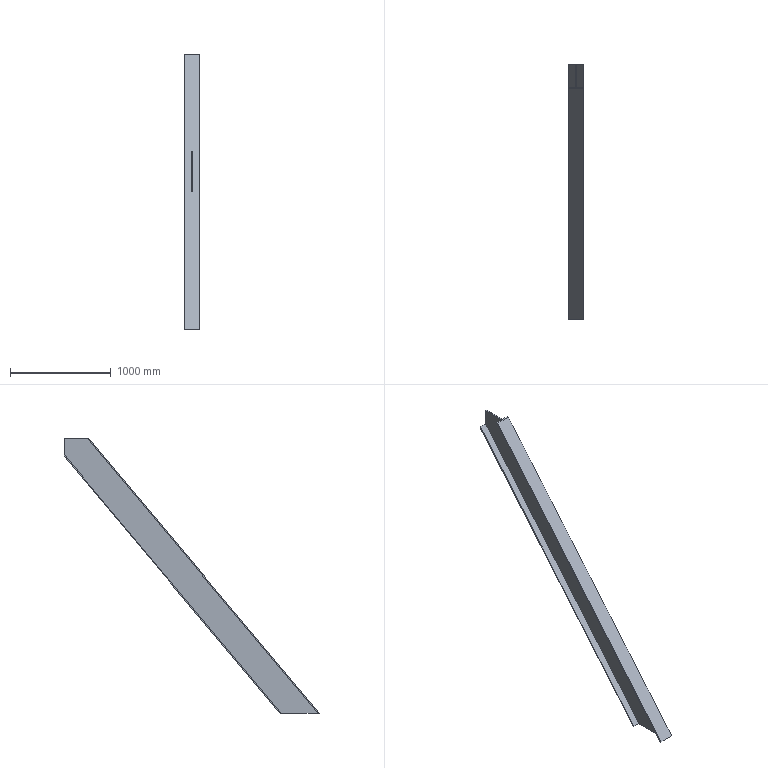Component | NX | ZHIJIA_XIE1 | 1 solid | 15 faces | box 150 x 2527.87 x 2724.41 mm | volume 20181722 mm3 | plane 15
STEP:
#1=CARTESIAN_POINT('',(0.,0.,0.));
#2=DIRECTION('',(0.,0.,1.));
#3=DIRECTION('',(1.,0.,0.));
#4=AXIS2_PLACEMENT_3D('',#1,#2,#3);
#5=CARTESIAN_POINT('',(2505.,2625.,3361.44));
#6=VERTEX_POINT('',#5);
#7=CARTESIAN_POINT('',(2505.,475.697,800.));
#8=VERTEX_POINT('',#7);
#9=CARTESIAN_POINT('',(2505.,2812.666,3585.092));
#10=DIRECTION('',(0.,-0.6428,-0.766));
#11=VECTOR('',#10,1.);
#12=LINE('',#9,#11);
#13=CARTESIAN_POINT('',(2505.,2598.174,3765.072));
#14=DIRECTION('',(-1.,0.,-0.));
#15=DIRECTION('',(-0.,-0.766,0.6428));
#16=AXIS2_PLACEMENT_3D('',#13,#14,#15);
#17=PLANE('',#16);
#18=CARTESIAN_POINT('',(-280.,-0.));
#19=DIRECTION('',(0.,-1.));
#20=VECTOR('',#19,1.);
#21=LINE('',#18,#20);
#22=(GEOMETRIC_REPRESENTATION_CONTEXT(2)PARAMETRIC_REPRESENTATION_CONTEXT()REPRESENTATION_CONTEXT('',''));
#23=DEFINITIONAL_REPRESENTATION('',(#21),#22);
#24=PCURVE('',#17,#23);
#25=CARTESIAN_POINT('',(2505.,2812.666,3585.092));
#26=DIRECTION('',(0.,0.766,-0.6428));
#27=DIRECTION('',(0.,0.6428,0.766));
#28=AXIS2_PLACEMENT_3D('',#25,#26,#27);
#29=PLANE('',#28);
#30=CARTESIAN_POINT('',(0.,0.));
#31=DIRECTION('',(-1.,0.));
#32=VECTOR('',#31,1.);
#33=LINE('',#30,#32);
#34=(GEOMETRIC_REPRESENTATION_CONTEXT(2)PARAMETRIC_REPRESENTATION_CONTEXT()REPRESENTATION_CONTEXT('',''));
#35=DEFINITIONAL_REPRESENTATION('',(#33),#34);
#36=PCURVE('',#29,#35);
#37=SURFACE_CURVE('',#12,(#24,#36),.PCURVE_S1.);
#38=EDGE_CURVE('',#6,#8,#37,.T.);
#39=ORIENTED_EDGE('',*,*,#38,.F.);
#40=CARTESIAN_POINT('',(2505.,2625.,3524.41));
#41=VERTEX_POINT('',#40);
#42=CARTESIAN_POINT('',(2505.,2625.,3765.072));
#43=DIRECTION('',(-0.,-0.,1.));
#44=VECTOR('',#43,1.);
#45=LINE('',#42,#44);
#46=CARTESIAN_POINT('',(-20.55,17.244));
#47=DIRECTION('',(0.6428,0.766));
#48=VECTOR('',#47,1.);
#49=LINE('',#46,#48);
#50=(GEOMETRIC_REPRESENTATION_CONTEXT(2)PARAMETRIC_REPRESENTATION_CONTEXT()REPRESENTATION_CONTEXT('',''));
#51=DEFINITIONAL_REPRESENTATION('',(#49),#50);
#52=PCURVE('',#17,#51);
#53=CARTESIAN_POINT('',(9500.,2625.,3117.693));
#54=DIRECTION('',(0.,-1.,-0.));
#55=DIRECTION('',(0.,0.,-1.));
#56=AXIS2_PLACEMENT_3D('',#53,#54,#55);
#57=PLANE('',#56);
#58=CARTESIAN_POINT('',(-647.379,-6995.));
#59=DIRECTION('',(-1.,-0.));
#60=VECTOR('',#59,1.);
#61=LINE('',#58,#60);
#62=(GEOMETRIC_REPRESENTATION_CONTEXT(2)PARAMETRIC_REPRESENTATION_CONTEXT()REPRESENTATION_CONTEXT('',''));
#63=DEFINITIONAL_REPRESENTATION('',(#61),#62);
#64=PCURVE('',#57,#63);
#65=SURFACE_CURVE('',#45,(#52,#64),.PCURVE_S1.);
#66=EDGE_CURVE('',#6,#41,#65,.T.);
#67=ORIENTED_EDGE('',*,*,#66,.T.);
#68=CARTESIAN_POINT('',(2505.,2396.234,3524.41));
#69=VERTEX_POINT('',#68);
#70=CARTESIAN_POINT('',(2505.,2598.174,3524.41));
#71=DIRECTION('',(-0.,-1.,0.));
#72=VECTOR('',#71,1.);
#73=LINE('',#70,#72);
#74=CARTESIAN_POINT('',(-154.695,-184.358));
#75=DIRECTION('',(0.766,-0.6428));
#76=VECTOR('',#75,1.);
#77=LINE('',#74,#76);
#78=(GEOMETRIC_REPRESENTATION_CONTEXT(2)PARAMETRIC_REPRESENTATION_CONTEXT()REPRESENTATION_CONTEXT('',''));
#79=DEFINITIONAL_REPRESENTATION('',(#77),#78);
#80=PCURVE('',#17,#79);
#81=CARTESIAN_POINT('',(9500.,2625.,3524.41));
#82=DIRECTION('',(0.,-0.,-1.));
#83=DIRECTION('',(0.,1.,-0.));
#84=AXIS2_PLACEMENT_3D('',#81,#82,#83);
#85=PLANE('',#84);
#86=CARTESIAN_POINT('',(-26.826,-6995.));
#87=DIRECTION('',(-1.,-0.));
#88=VECTOR('',#87,1.);
#89=LINE('',#86,#88);
#90=(GEOMETRIC_REPRESENTATION_CONTEXT(2)PARAMETRIC_REPRESENTATION_CONTEXT()REPRESENTATION_CONTEXT('',''));
#91=DEFINITIONAL_REPRESENTATION('',(#89),#90);
#92=PCURVE('',#85,#91);
#93=SURFACE_CURVE('',#73,(#80,#92),.PCURVE_S1.);
#94=EDGE_CURVE('',#41,#69,#93,.T.);
#95=ORIENTED_EDGE('',*,*,#94,.T.);
#96=CARTESIAN_POINT('',(2505.,110.183,800.));
#97=VERTEX_POINT('',#96);
#98=CARTESIAN_POINT('',(2505.,2598.174,3765.072));
#99=DIRECTION('',(0.,-0.6428,-0.766));
#100=VECTOR('',#99,1.);
#101=LINE('',#98,#100);
#102=CARTESIAN_POINT('',(0.,0.));
#103=DIRECTION('',(0.,-1.));
#104=VECTOR('',#103,1.);
#105=LINE('',#102,#104);
#106=(GEOMETRIC_REPRESENTATION_CONTEXT(2)PARAMETRIC_REPRESENTATION_CONTEXT()REPRESENTATION_CONTEXT('',''));
#107=DEFINITIONAL_REPRESENTATION('',(#105),#106);
#108=PCURVE('',#17,#107);
#109=CARTESIAN_POINT('',(2575.,2598.174,3765.072));
#110=DIRECTION('',(0.,-0.766,0.6428));
#111=DIRECTION('',(0.,-0.6428,-0.766));
#112=AXIS2_PLACEMENT_3D('',#109,#110,#111);
#113=PLANE('',#112);
#114=CARTESIAN_POINT('',(0.,-70.));
#115=DIRECTION('',(1.,0.));
#116=VECTOR('',#115,1.);
#117=LINE('',#114,#116);
#118=(GEOMETRIC_REPRESENTATION_CONTEXT(2)PARAMETRIC_REPRESENTATION_CONTEXT()REPRESENTATION_CONTEXT('',''));
#119=DEFINITIONAL_REPRESENTATION('',(#117),#118);
#120=PCURVE('',#113,#119);
#121=SURFACE_CURVE('',#101,(#108,#120),.PCURVE_S1.);
#122=EDGE_CURVE('',#69,#97,#121,.T.);
#123=ORIENTED_EDGE('',*,*,#122,.T.);
#124=CARTESIAN_POINT('',(2505.,2598.174,800.));
#125=DIRECTION('',(-0.,-1.,-0.));
#126=VECTOR('',#125,1.);
#127=LINE('',#124,#126);
#128=CARTESIAN_POINT('',(-1905.912,-2271.377));
#129=DIRECTION('',(0.766,-0.6428));
#130=VECTOR('',#129,1.);
#131=LINE('',#128,#130);
#132=(GEOMETRIC_REPRESENTATION_CONTEXT(2)PARAMETRIC_REPRESENTATION_CONTEXT()REPRESENTATION_CONTEXT('',''));
#133=DEFINITIONAL_REPRESENTATION('',(#131),#132);
#134=PCURVE('',#17,#133);
#135=CARTESIAN_POINT('',(9500.,631.661,800.));
#136=DIRECTION('',(0.,0.,-1.));
#137=DIRECTION('',(0.,1.,0.));
#138=AXIS2_PLACEMENT_3D('',#135,#136,#137);
#139=PLANE('',#138);
#140=CARTESIAN_POINT('',(1966.512,-6995.));
#141=DIRECTION('',(-1.,-0.));
#142=VECTOR('',#141,1.);
#143=LINE('',#140,#142);
#144=(GEOMETRIC_REPRESENTATION_CONTEXT(2)PARAMETRIC_REPRESENTATION_CONTEXT()REPRESENTATION_CONTEXT('',''));
#145=DEFINITIONAL_REPRESENTATION('',(#143),#144);
#146=PCURVE('',#139,#145);
#147=SURFACE_CURVE('',#127,(#134,#146),.PCURVE_S1.);
#148=EDGE_CURVE('',#8,#97,#147,.T.);
#149=ORIENTED_EDGE('',*,*,#148,.F.);
#150=EDGE_LOOP('',(#39,#67,#95,#123,#149));
#151=FACE_BOUND('',#150,.T.);
#152=ADVANCED_FACE('',(#151),#17,.F.);
#153=CARTESIAN_POINT('',(2575.,2625.,3361.44));
#154=VERTEX_POINT('',#153);
#155=CARTESIAN_POINT('',(2575.,475.697,800.));
#156=VERTEX_POINT('',#155);
#157=CARTESIAN_POINT('',(2575.,2812.666,3585.092));
#158=DIRECTION('',(0.,-0.6428,-0.766));
#159=VECTOR('',#158,1.);
#160=LINE('',#157,#159);
#161=CARTESIAN_POINT('',(0.,70.));
#162=DIRECTION('',(-1.,0.));
#163=VECTOR('',#162,1.);
#164=LINE('',#161,#163);
#165=(GEOMETRIC_REPRESENTATION_CONTEXT(2)PARAMETRIC_REPRESENTATION_CONTEXT()REPRESENTATION_CONTEXT('',''));
#166=DEFINITIONAL_REPRESENTATION('',(#164),#165);
#167=PCURVE('',#29,#166);
#168=CARTESIAN_POINT('',(2575.,2812.666,3585.092));
#169=DIRECTION('',(-1.,0.,-0.));
#170=DIRECTION('',(-0.,-0.766,0.6428));
#171=AXIS2_PLACEMENT_3D('',#168,#169,#170);
#172=PLANE('',#171);
#173=CARTESIAN_POINT('',(0.,0.));
#174=DIRECTION('',(0.,-1.));
#175=VECTOR('',#174,1.);
#176=LINE('',#173,#175);
#177=(GEOMETRIC_REPRESENTATION_CONTEXT(2)PARAMETRIC_REPRESENTATION_CONTEXT()REPRESENTATION_CONTEXT('',''));
#178=DEFINITIONAL_REPRESENTATION('',(#176),#177);
#179=PCURVE('',#172,#178);
#180=SURFACE_CURVE('',#160,(#167,#179),.PCURVE_S1.);
#181=EDGE_CURVE('',#154,#156,#180,.T.);
#182=ORIENTED_EDGE('',*,*,#181,.F.);
#183=CARTESIAN_POINT('',(2505.,2625.,3361.44));
#184=DIRECTION('',(-1.,0.,0.));
#185=VECTOR('',#184,1.);
#186=LINE('',#183,#185);
#187=CARTESIAN_POINT('',(-291.957,0.));
#188=DIRECTION('',(0.,-1.));
#189=VECTOR('',#188,1.);
#190=LINE('',#187,#189);
#191=(GEOMETRIC_REPRESENTATION_CONTEXT(2)PARAMETRIC_REPRESENTATION_CONTEXT()REPRESENTATION_CONTEXT('',''));
#192=DEFINITIONAL_REPRESENTATION('',(#190),#191);
#193=PCURVE('',#29,#192);
#194=CARTESIAN_POINT('',(-243.747,-6995.));
#195=DIRECTION('',(0.,-1.));
#196=VECTOR('',#195,1.);
#197=LINE('',#194,#196);
#198=(GEOMETRIC_REPRESENTATION_CONTEXT(2)PARAMETRIC_REPRESENTATION_CONTEXT()REPRESENTATION_CONTEXT('',''));
#199=DEFINITIONAL_REPRESENTATION('',(#197),#198);
#200=PCURVE('',#57,#199);
#201=SURFACE_CURVE('',#186,(#193,#200),.PCURVE_S1.);
#202=EDGE_CURVE('',#154,#6,#201,.T.);
#203=ORIENTED_EDGE('',*,*,#202,.T.);
#204=ORIENTED_EDGE('',*,*,#38,.T.);
#205=CARTESIAN_POINT('',(2505.,475.697,800.));
#206=DIRECTION('',(-1.,0.,0.));
#207=VECTOR('',#206,1.);
#208=LINE('',#205,#207);
#209=CARTESIAN_POINT('',(-3635.679,0.));
#210=DIRECTION('',(0.,-1.));
#211=VECTOR('',#210,1.);
#212=LINE('',#209,#211);
#213=(GEOMETRIC_REPRESENTATION_CONTEXT(2)PARAMETRIC_REPRESENTATION_CONTEXT()REPRESENTATION_CONTEXT('',''));
#214=DEFINITIONAL_REPRESENTATION('',(#212),#213);
#215=PCURVE('',#29,#214);
#216=CARTESIAN_POINT('',(-155.965,-6995.));
#217=DIRECTION('',(0.,-1.));
#218=VECTOR('',#217,1.);
#219=LINE('',#216,#218);
#220=(GEOMETRIC_REPRESENTATION_CONTEXT(2)PARAMETRIC_REPRESENTATION_CONTEXT()REPRESENTATION_CONTEXT('',''));
#221=DEFINITIONAL_REPRESENTATION('',(#219),#220);
#222=PCURVE('',#139,#221);
#223=SURFACE_CURVE('',#208,(#215,#222),.PCURVE_S1.);
#224=EDGE_CURVE('',#156,#8,#223,.T.);
#225=ORIENTED_EDGE('',*,*,#224,.F.);
#226=EDGE_LOOP('',(#182,#203,#204,#225));
#227=FACE_BOUND('',#226,.T.);
#228=ADVANCED_FACE('',(#227),#29,.F.);
#229=CARTESIAN_POINT('',(2575.,2625.,3345.883));
#230=VERTEX_POINT('',#229);
#231=CARTESIAN_POINT('',(2575.,488.751,800.));
#232=VERTEX_POINT('',#231);
#233=CARTESIAN_POINT('',(2575.,2820.327,3578.664));
#234=DIRECTION('',(0.,-0.6428,-0.766));
#235=VECTOR('',#234,1.);
#236=LINE('',#233,#235);
#237=CARTESIAN_POINT('',(-10.,0.));
#238=DIRECTION('',(0.,-1.));
#239=VECTOR('',#238,1.);
#240=LINE('',#237,#239);
#241=(GEOMETRIC_REPRESENTATION_CONTEXT(2)PARAMETRIC_REPRESENTATION_CONTEXT()REPRESENTATION_CONTEXT('',''));
#242=DEFINITIONAL_REPRESENTATION('',(#240),#241);
#243=PCURVE('',#172,#242);
#244=CARTESIAN_POINT('',(2575.,2820.327,3578.664));
#245=DIRECTION('',(0.,-0.766,0.6428));
#246=DIRECTION('',(0.,-0.6428,-0.766));
#247=AXIS2_PLACEMENT_3D('',#244,#245,#246);
#248=PLANE('',#247);
#249=CARTESIAN_POINT('',(0.,0.));
#250=DIRECTION('',(1.,0.));
#251=VECTOR('',#250,1.);
#252=LINE('',#249,#251);
#253=(GEOMETRIC_REPRESENTATION_CONTEXT(2)PARAMETRIC_REPRESENTATION_CONTEXT()REPRESENTATION_CONTEXT('',''));
#254=DEFINITIONAL_REPRESENTATION('',(#252),#253);
#255=PCURVE('',#248,#254);
#256=SURFACE_CURVE('',#236,(#243,#255),.PCURVE_S1.);
#257=EDGE_CURVE('',#230,#232,#256,.T.);
#258=ORIENTED_EDGE('',*,*,#257,.F.);
#259=CARTESIAN_POINT('',(2575.,2625.,3585.092));
#260=DIRECTION('',(-0.,-0.,1.));
#261=VECTOR('',#260,1.);
#262=LINE('',#259,#261);
#263=CARTESIAN_POINT('',(143.761,-120.63));
#264=DIRECTION('',(0.6428,0.766));
#265=VECTOR('',#264,1.);
#266=LINE('',#263,#265);
#267=(GEOMETRIC_REPRESENTATION_CONTEXT(2)PARAMETRIC_REPRESENTATION_CONTEXT()REPRESENTATION_CONTEXT('',''));
#268=DEFINITIONAL_REPRESENTATION('',(#266),#267);
#269=PCURVE('',#172,#268);
#270=CARTESIAN_POINT('',(-467.399,-6925.));
#271=DIRECTION('',(-1.,-0.));
#272=VECTOR('',#271,1.);
#273=LINE('',#270,#272);
#274=(GEOMETRIC_REPRESENTATION_CONTEXT(2)PARAMETRIC_REPRESENTATION_CONTEXT()REPRESENTATION_CONTEXT('',''));
#275=DEFINITIONAL_REPRESENTATION('',(#273),#274);
#276=PCURVE('',#57,#275);
#277=SURFACE_CURVE('',#262,(#269,#276),.PCURVE_S1.);
#278=EDGE_CURVE('',#230,#154,#277,.T.);
#279=ORIENTED_EDGE('',*,*,#278,.T.);
#280=ORIENTED_EDGE('',*,*,#181,.T.);
#281=CARTESIAN_POINT('',(2575.,2812.666,800.));
#282=DIRECTION('',(-0.,-1.,-0.));
#283=VECTOR('',#282,1.);
#284=LINE('',#281,#283);
#285=CARTESIAN_POINT('',(-1790.223,-2133.504));
#286=DIRECTION('',(0.766,-0.6428));
#287=VECTOR('',#286,1.);
#288=LINE('',#285,#287);
#289=(GEOMETRIC_REPRESENTATION_CONTEXT(2)PARAMETRIC_REPRESENTATION_CONTEXT()REPRESENTATION_CONTEXT('',''));
#290=DEFINITIONAL_REPRESENTATION('',(#288),#289);
#291=PCURVE('',#172,#290);
#292=CARTESIAN_POINT('',(2181.005,-6925.));
#293=DIRECTION('',(-1.,-0.));
#294=VECTOR('',#293,1.);
#295=LINE('',#292,#294);
#296=(GEOMETRIC_REPRESENTATION_CONTEXT(2)PARAMETRIC_REPRESENTATION_CONTEXT()REPRESENTATION_CONTEXT('',''));
#297=DEFINITIONAL_REPRESENTATION('',(#295),#296);
#298=PCURVE('',#139,#297);
#299=SURFACE_CURVE('',#284,(#291,#298),.PCURVE_S1.);
#300=EDGE_CURVE('',#232,#156,#299,.T.);
#301=ORIENTED_EDGE('',*,*,#300,.F.);
#302=EDGE_LOOP('',(#258,#279,#280,#301));
#303=FACE_BOUND('',#302,.T.);
#304=ADVANCED_FACE('',(#303),#172,.F.);
#305=CARTESIAN_POINT('',(2425.,2625.,3345.883));
#306=VERTEX_POINT('',#305);
#307=CARTESIAN_POINT('',(2425.,488.751,800.));
#308=VERTEX_POINT('',#307);
#309=CARTESIAN_POINT('',(2425.,2820.327,3578.664));
#310=DIRECTION('',(0.,-0.6428,-0.766));
#311=VECTOR('',#310,1.);
#312=LINE('',#309,#311);
#313=CARTESIAN_POINT('',(0.,-150.));
#314=DIRECTION('',(1.,0.));
#315=VECTOR('',#314,1.);
#316=LINE('',#313,#315);
#317=(GEOMETRIC_REPRESENTATION_CONTEXT(2)PARAMETRIC_REPRESENTATION_CONTEXT()REPRESENTATION_CONTEXT('',''));
#318=DEFINITIONAL_REPRESENTATION('',(#316),#317);
#319=PCURVE('',#248,#318);
#320=CARTESIAN_POINT('',(2425.,2820.327,3578.664));
#321=DIRECTION('',(1.,-0.,0.));
#322=DIRECTION('',(0.,0.766,-0.6428));
#323=AXIS2_PLACEMENT_3D('',#320,#321,#322);
#324=PLANE('',#323);
#325=CARTESIAN_POINT('',(0.,0.));
#326=DIRECTION('',(0.,-1.));
#327=VECTOR('',#326,1.);
#328=LINE('',#325,#327);
#329=(GEOMETRIC_REPRESENTATION_CONTEXT(2)PARAMETRIC_REPRESENTATION_CONTEXT()REPRESENTATION_CONTEXT('',''));
#330=DEFINITIONAL_REPRESENTATION('',(#328),#329);
#331=PCURVE('',#324,#330);
#332=SURFACE_CURVE('',#312,(#319,#331),.PCURVE_S1.);
#333=EDGE_CURVE('',#306,#308,#332,.T.);
#334=ORIENTED_EDGE('',*,*,#333,.F.);
#335=CARTESIAN_POINT('',(2575.,2625.,3345.883));
#336=DIRECTION('',(1.,0.,0.));
#337=VECTOR('',#336,1.);
#338=LINE('',#335,#337);
#339=CARTESIAN_POINT('',(303.874,0.));
#340=DIRECTION('',(0.,1.));
#341=VECTOR('',#340,1.);
#342=LINE('',#339,#341);
#343=(GEOMETRIC_REPRESENTATION_CONTEXT(2)PARAMETRIC_REPRESENTATION_CONTEXT()REPRESENTATION_CONTEXT('',''));
#344=DEFINITIONAL_REPRESENTATION('',(#342),#343);
#345=PCURVE('',#248,#344);
#346=CARTESIAN_POINT('',(-228.19,-6925.));
#347=DIRECTION('',(0.,1.));
#348=VECTOR('',#347,1.);
#349=LINE('',#346,#348);
#350=(GEOMETRIC_REPRESENTATION_CONTEXT(2)PARAMETRIC_REPRESENTATION_CONTEXT()REPRESENTATION_CONTEXT('',''));
#351=DEFINITIONAL_REPRESENTATION('',(#349),#350);
#352=PCURVE('',#57,#351);
#353=SURFACE_CURVE('',#338,(#345,#352),.PCURVE_S1.);
#354=EDGE_CURVE('',#306,#230,#353,.T.);
#355=ORIENTED_EDGE('',*,*,#354,.T.);
#356=ORIENTED_EDGE('',*,*,#257,.T.);
#357=CARTESIAN_POINT('',(2575.,488.751,800.));
#358=DIRECTION('',(1.,0.,0.));
#359=VECTOR('',#358,1.);
#360=LINE('',#357,#359);
#361=CARTESIAN_POINT('',(3627.288,0.));
#362=DIRECTION('',(0.,1.));
#363=VECTOR('',#362,1.);
#364=LINE('',#361,#363);
#365=(GEOMETRIC_REPRESENTATION_CONTEXT(2)PARAMETRIC_REPRESENTATION_CONTEXT()REPRESENTATION_CONTEXT('',''));
#366=DEFINITIONAL_REPRESENTATION('',(#364),#365);
#367=PCURVE('',#248,#366);
#368=CARTESIAN_POINT('',(-142.911,-6925.));
#369=DIRECTION('',(0.,1.));
#370=VECTOR('',#369,1.);
#371=LINE('',#368,#370);
#372=(GEOMETRIC_REPRESENTATION_CONTEXT(2)PARAMETRIC_REPRESENTATION_CONTEXT()REPRESENTATION_CONTEXT('',''));
#373=DEFINITIONAL_REPRESENTATION('',(#371),#372);
#374=PCURVE('',#139,#373);
#375=SURFACE_CURVE('',#360,(#367,#374),.PCURVE_S1.);
#376=EDGE_CURVE('',#308,#232,#375,.T.);
#377=ORIENTED_EDGE('',*,*,#376,.F.);
#378=EDGE_LOOP('',(#334,#355,#356,#377));
#379=FACE_BOUND('',#378,.T.);
#380=ADVANCED_FACE('',(#379),#248,.F.);
#381=CARTESIAN_POINT('',(2425.,2625.,3361.44));
#382=VERTEX_POINT('',#381);
#383=CARTESIAN_POINT('',(2425.,475.697,800.));
#384=VERTEX_POINT('',#383);
#385=CARTESIAN_POINT('',(2425.,2812.666,3585.092));
#386=DIRECTION('',(0.,-0.6428,-0.766));
#387=VECTOR('',#386,1.);
#388=LINE('',#385,#387);
#389=CARTESIAN_POINT('',(-10.,-0.));
#390=DIRECTION('',(0.,-1.));
#391=VECTOR('',#390,1.);
#392=LINE('',#389,#391);
#393=(GEOMETRIC_REPRESENTATION_CONTEXT(2)PARAMETRIC_REPRESENTATION_CONTEXT()REPRESENTATION_CONTEXT('',''));
#394=DEFINITIONAL_REPRESENTATION('',(#392),#393);
#395=PCURVE('',#324,#394);
#396=CARTESIAN_POINT('',(2425.,2812.666,3585.092));
#397=DIRECTION('',(0.,0.766,-0.6428));
#398=DIRECTION('',(0.,0.6428,0.766));
#399=AXIS2_PLACEMENT_3D('',#396,#397,#398);
#400=PLANE('',#399);
#401=CARTESIAN_POINT('',(0.,0.));
#402=DIRECTION('',(-1.,0.));
#403=VECTOR('',#402,1.);
#404=LINE('',#401,#403);
#405=(GEOMETRIC_REPRESENTATION_CONTEXT(2)PARAMETRIC_REPRESENTATION_CONTEXT()REPRESENTATION_CONTEXT('',''));
#406=DEFINITIONAL_REPRESENTATION('',(#404),#405);
#407=PCURVE('',#400,#406);
#408=SURFACE_CURVE('',#388,(#395,#407),.PCURVE_S1.);
#409=EDGE_CURVE('',#382,#384,#408,.T.);
#410=ORIENTED_EDGE('',*,*,#409,.F.);
#411=CARTESIAN_POINT('',(2425.,2625.,3578.664));
#412=DIRECTION('',(0.,0.,-1.));
#413=VECTOR('',#412,1.);
#414=LINE('',#411,#413);
#415=CARTESIAN_POINT('',(-149.629,-125.554));
#416=DIRECTION('',(0.6428,-0.766));
#417=VECTOR('',#416,1.);
#418=LINE('',#415,#417);
#419=(GEOMETRIC_REPRESENTATION_CONTEXT(2)PARAMETRIC_REPRESENTATION_CONTEXT()REPRESENTATION_CONTEXT('',''));
#420=DEFINITIONAL_REPRESENTATION('',(#418),#419);
#421=PCURVE('',#324,#420);
#422=CARTESIAN_POINT('',(-460.971,-7075.));
#423=DIRECTION('',(1.,0.));
#424=VECTOR('',#423,1.);
#425=LINE('',#422,#424);
#426=(GEOMETRIC_REPRESENTATION_CONTEXT(2)PARAMETRIC_REPRESENTATION_CONTEXT()REPRESENTATION_CONTEXT('',''));
#427=DEFINITIONAL_REPRESENTATION('',(#425),#426);
#428=PCURVE('',#57,#427);
#429=SURFACE_CURVE('',#414,(#421,#428),.PCURVE_S1.);
#430=EDGE_CURVE('',#382,#306,#429,.T.);
#431=ORIENTED_EDGE('',*,*,#430,.T.);
#432=ORIENTED_EDGE('',*,*,#333,.T.);
#433=CARTESIAN_POINT('',(2425.,2820.327,800.));
#434=DIRECTION('',(0.,1.,0.));
#435=VECTOR('',#434,1.);
#436=LINE('',#433,#435);
#437=CARTESIAN_POINT('',(1786.091,-2128.58));
#438=DIRECTION('',(0.766,0.6428));
#439=VECTOR('',#438,1.);
#440=LINE('',#437,#439);
#441=(GEOMETRIC_REPRESENTATION_CONTEXT(2)PARAMETRIC_REPRESENTATION_CONTEXT()REPRESENTATION_CONTEXT('',''));
#442=DEFINITIONAL_REPRESENTATION('',(#440),#441);
#443=PCURVE('',#324,#442);
#444=CARTESIAN_POINT('',(2188.665,-7075.));
#445=DIRECTION('',(1.,0.));
#446=VECTOR('',#445,1.);
#447=LINE('',#444,#446);
#448=(GEOMETRIC_REPRESENTATION_CONTEXT(2)PARAMETRIC_REPRESENTATION_CONTEXT()REPRESENTATION_CONTEXT('',''));
#449=DEFINITIONAL_REPRESENTATION('',(#447),#448);
#450=PCURVE('',#139,#449);
#451=SURFACE_CURVE('',#436,(#443,#450),.PCURVE_S1.);
#452=EDGE_CURVE('',#384,#308,#451,.T.);
#453=ORIENTED_EDGE('',*,*,#452,.F.);
#454=EDGE_LOOP('',(#410,#431,#432,#453));
#455=FACE_BOUND('',#454,.T.);
#456=ADVANCED_FACE('',(#455),#324,.F.);
#457=CARTESIAN_POINT('',(2495.,2625.,3361.44));
#458=VERTEX_POINT('',#457);
#459=CARTESIAN_POINT('',(2495.,475.697,800.));
#460=VERTEX_POINT('',#459);
#461=CARTESIAN_POINT('',(2495.,2812.666,3585.092));
#462=DIRECTION('',(0.,-0.6428,-0.766));
#463=VECTOR('',#462,1.);
#464=LINE('',#461,#463);
#465=CARTESIAN_POINT('',(0.,70.));
#466=DIRECTION('',(-1.,0.));
#467=VECTOR('',#466,1.);
#468=LINE('',#465,#467);
#469=(GEOMETRIC_REPRESENTATION_CONTEXT(2)PARAMETRIC_REPRESENTATION_CONTEXT()REPRESENTATION_CONTEXT('',''));
#470=DEFINITIONAL_REPRESENTATION('',(#468),#469);
#471=PCURVE('',#400,#470);
#472=CARTESIAN_POINT('',(2495.,2812.666,3585.092));
#473=DIRECTION('',(1.,-0.,0.));
#474=DIRECTION('',(0.,0.766,-0.6428));
#475=AXIS2_PLACEMENT_3D('',#472,#473,#474);
#476=PLANE('',#475);
#477=CARTESIAN_POINT('',(0.,0.));
#478=DIRECTION('',(0.,-1.));
#479=VECTOR('',#478,1.);
#480=LINE('',#477,#479);
#481=(GEOMETRIC_REPRESENTATION_CONTEXT(2)PARAMETRIC_REPRESENTATION_CONTEXT()REPRESENTATION_CONTEXT('',''));
#482=DEFINITIONAL_REPRESENTATION('',(#480),#481);
#483=PCURVE('',#476,#482);
#484=SURFACE_CURVE('',#464,(#471,#483),.PCURVE_S1.);
#485=EDGE_CURVE('',#458,#460,#484,.T.);
#486=ORIENTED_EDGE('',*,*,#485,.F.);
#487=CARTESIAN_POINT('',(2425.,2625.,3361.44));
#488=DIRECTION('',(-1.,0.,0.));
#489=VECTOR('',#488,1.);
#490=LINE('',#487,#489);
#491=CARTESIAN_POINT('',(-291.957,0.));
#492=DIRECTION('',(0.,-1.));
#493=VECTOR('',#492,1.);
#494=LINE('',#491,#493);
#495=(GEOMETRIC_REPRESENTATION_CONTEXT(2)PARAMETRIC_REPRESENTATION_CONTEXT()REPRESENTATION_CONTEXT('',''));
#496=DEFINITIONAL_REPRESENTATION('',(#494),#495);
#497=PCURVE('',#400,#496);
#498=CARTESIAN_POINT('',(-243.747,-7075.));
#499=DIRECTION('',(0.,-1.));
#500=VECTOR('',#499,1.);
#501=LINE('',#498,#500);
#502=(GEOMETRIC_REPRESENTATION_CONTEXT(2)PARAMETRIC_REPRESENTATION_CONTEXT()REPRESENTATION_CONTEXT('',''));
#503=DEFINITIONAL_REPRESENTATION('',(#501),#502);
#504=PCURVE('',#57,#503);
#505=SURFACE_CURVE('',#490,(#497,#504),.PCURVE_S1.);
#506=EDGE_CURVE('',#458,#382,#505,.T.);
#507=ORIENTED_EDGE('',*,*,#506,.T.);
#508=ORIENTED_EDGE('',*,*,#409,.T.);
#509=CARTESIAN_POINT('',(2425.,475.697,800.));
#510=DIRECTION('',(-1.,0.,0.));
#511=VECTOR('',#510,1.);
#512=LINE('',#509,#511);
#513=CARTESIAN_POINT('',(-3635.679,0.));
#514=DIRECTION('',(0.,-1.));
#515=VECTOR('',#514,1.);
#516=LINE('',#513,#515);
#517=(GEOMETRIC_REPRESENTATION_CONTEXT(2)PARAMETRIC_REPRESENTATION_CONTEXT()REPRESENTATION_CONTEXT('',''));
#518=DEFINITIONAL_REPRESENTATION('',(#516),#517);
#519=PCURVE('',#400,#518);
#520=CARTESIAN_POINT('',(-155.965,-7075.));
#521=DIRECTION('',(0.,-1.));
#522=VECTOR('',#521,1.);
#523=LINE('',#520,#522);
#524=(GEOMETRIC_REPRESENTATION_CONTEXT(2)PARAMETRIC_REPRESENTATION_CONTEXT()REPRESENTATION_CONTEXT('',''));
#525=DEFINITIONAL_REPRESENTATION('',(#523),#524);
#526=PCURVE('',#139,#525);
#527=SURFACE_CURVE('',#512,(#519,#526),.PCURVE_S1.);
#528=EDGE_CURVE('',#460,#384,#527,.T.);
#529=ORIENTED_EDGE('',*,*,#528,.F.);
#530=EDGE_LOOP('',(#486,#507,#508,#529));
#531=FACE_BOUND('',#530,.T.);
#532=ADVANCED_FACE('',(#531),#400,.F.);
#533=CARTESIAN_POINT('',(2495.,2396.234,3524.41));
#534=VERTEX_POINT('',#533);
#535=CARTESIAN_POINT('',(2495.,2625.,3524.41));
#536=VERTEX_POINT('',#535);
#537=CARTESIAN_POINT('',(2495.,2812.666,3524.41));
#538=DIRECTION('',(0.,1.,-0.));
#539=VECTOR('',#538,1.);
#540=LINE('',#537,#539);
#541=CARTESIAN_POINT('',(39.005,-46.485));
#542=DIRECTION('',(0.766,0.6428));
#543=VECTOR('',#542,1.);
#544=LINE('',#541,#543);
#545=(GEOMETRIC_REPRESENTATION_CONTEXT(2)PARAMETRIC_REPRESENTATION_CONTEXT()REPRESENTATION_CONTEXT('',''));
#546=DEFINITIONAL_REPRESENTATION('',(#544),#545);
#547=PCURVE('',#476,#546);
#548=CARTESIAN_POINT('',(187.666,-7005.));
#549=DIRECTION('',(1.,0.));
#550=VECTOR('',#549,1.);
#551=LINE('',#548,#550);
#552=(GEOMETRIC_REPRESENTATION_CONTEXT(2)PARAMETRIC_REPRESENTATION_CONTEXT()REPRESENTATION_CONTEXT('',''));
#553=DEFINITIONAL_REPRESENTATION('',(#551),#552);
#554=PCURVE('',#85,#553);
#555=SURFACE_CURVE('',#540,(#547,#554),.PCURVE_S1.);
#556=EDGE_CURVE('',#534,#536,#555,.T.);
#557=ORIENTED_EDGE('',*,*,#556,.T.);
#558=CARTESIAN_POINT('',(2495.,2625.,3585.092));
#559=DIRECTION('',(0.,0.,-1.));
#560=VECTOR('',#559,1.);
#561=LINE('',#558,#560);
#562=CARTESIAN_POINT('',(-143.761,-120.63));
#563=DIRECTION('',(0.6428,-0.766));
#564=VECTOR('',#563,1.);
#565=LINE('',#562,#564);
#566=(GEOMETRIC_REPRESENTATION_CONTEXT(2)PARAMETRIC_REPRESENTATION_CONTEXT()REPRESENTATION_CONTEXT('',''));
#567=DEFINITIONAL_REPRESENTATION('',(#565),#566);
#568=PCURVE('',#476,#567);
#569=CARTESIAN_POINT('',(-467.399,-7005.));
#570=DIRECTION('',(1.,0.));
#571=VECTOR('',#570,1.);
#572=LINE('',#569,#571);
#573=(GEOMETRIC_REPRESENTATION_CONTEXT(2)PARAMETRIC_REPRESENTATION_CONTEXT()REPRESENTATION_CONTEXT('',''));
#574=DEFINITIONAL_REPRESENTATION('',(#572),#573);
#575=PCURVE('',#57,#574);
#576=SURFACE_CURVE('',#561,(#568,#575),.PCURVE_S1.);
#577=EDGE_CURVE('',#536,#458,#576,.T.);
#578=ORIENTED_EDGE('',*,*,#577,.T.);
#579=ORIENTED_EDGE('',*,*,#485,.T.);
#580=CARTESIAN_POINT('',(2495.,110.183,800.));
#581=VERTEX_POINT('',#580);
#582=CARTESIAN_POINT('',(2495.,2812.666,800.));
#583=DIRECTION('',(0.,1.,0.));
#584=VECTOR('',#583,1.);
#585=LINE('',#582,#584);
#586=CARTESIAN_POINT('',(1790.223,-2133.504));
#587=DIRECTION('',(0.766,0.6428));
#588=VECTOR('',#587,1.);
#589=LINE('',#586,#588);
#590=(GEOMETRIC_REPRESENTATION_CONTEXT(2)PARAMETRIC_REPRESENTATION_CONTEXT()REPRESENTATION_CONTEXT('',''));
#591=DEFINITIONAL_REPRESENTATION('',(#589),#590);
#592=PCURVE('',#476,#591);
#593=CARTESIAN_POINT('',(2181.005,-7005.));
#594=DIRECTION('',(1.,0.));
#595=VECTOR('',#594,1.);
#596=LINE('',#593,#595);
#597=(GEOMETRIC_REPRESENTATION_CONTEXT(2)PARAMETRIC_REPRESENTATION_CONTEXT()REPRESENTATION_CONTEXT('',''));
#598=DEFINITIONAL_REPRESENTATION('',(#596),#597);
#599=PCURVE('',#139,#598);
#600=SURFACE_CURVE('',#585,(#592,#599),.PCURVE_S1.);
#601=EDGE_CURVE('',#581,#460,#600,.T.);
#602=ORIENTED_EDGE('',*,*,#601,.F.);
#603=CARTESIAN_POINT('',(2495.,2598.174,3765.072));
#604=DIRECTION('',(0.,-0.6428,-0.766));
#605=VECTOR('',#604,1.);
#606=LINE('',#603,#605);
#607=CARTESIAN_POINT('',(-280.,0.));
#608=DIRECTION('',(0.,-1.));
#609=VECTOR('',#608,1.);
#610=LINE('',#607,#609);
#611=(GEOMETRIC_REPRESENTATION_CONTEXT(2)PARAMETRIC_REPRESENTATION_CONTEXT()REPRESENTATION_CONTEXT('',''));
#612=DEFINITIONAL_REPRESENTATION('',(#610),#611);
#613=PCURVE('',#476,#612);
#614=CARTESIAN_POINT('',(2495.,2598.174,3765.072));
#615=DIRECTION('',(0.,-0.766,0.6428));
#616=DIRECTION('',(0.,-0.6428,-0.766));
#617=AXIS2_PLACEMENT_3D('',#614,#615,#616);
#618=PLANE('',#617);
#619=CARTESIAN_POINT('',(0.,0.));
#620=DIRECTION('',(1.,0.));
#621=VECTOR('',#620,1.);
#622=LINE('',#619,#621);
#623=(GEOMETRIC_REPRESENTATION_CONTEXT(2)PARAMETRIC_REPRESENTATION_CONTEXT()REPRESENTATION_CONTEXT('',''));
#624=DEFINITIONAL_REPRESENTATION('',(#622),#623);
#625=PCURVE('',#618,#624);
#626=SURFACE_CURVE('',#606,(#613,#625),.PCURVE_S1.);
#627=EDGE_CURVE('',#534,#581,#626,.T.);
#628=ORIENTED_EDGE('',*,*,#627,.F.);
#629=EDGE_LOOP('',(#557,#578,#579,#602,#628));
#630=FACE_BOUND('',#629,.T.);
#631=ADVANCED_FACE('',(#630),#476,.F.);
#632=CARTESIAN_POINT('',(2425.,2396.234,3524.41));
#633=VERTEX_POINT('',#632);
#634=CARTESIAN_POINT('',(2425.,110.183,800.));
#635=VERTEX_POINT('',#634);
#636=CARTESIAN_POINT('',(2425.,2598.174,3765.072));
#637=DIRECTION('',(0.,-0.6428,-0.766));
#638=VECTOR('',#637,1.);
#639=LINE('',#636,#638);
#640=CARTESIAN_POINT('',(0.,-70.));
#641=DIRECTION('',(1.,0.));
#642=VECTOR('',#641,1.);
#643=LINE('',#640,#642);
#644=(GEOMETRIC_REPRESENTATION_CONTEXT(2)PARAMETRIC_REPRESENTATION_CONTEXT()REPRESENTATION_CONTEXT('',''));
#645=DEFINITIONAL_REPRESENTATION('',(#643),#644);
#646=PCURVE('',#618,#645);
#647=CARTESIAN_POINT('',(2425.,2598.174,3765.072));
#648=DIRECTION('',(1.,-0.,0.));
#649=DIRECTION('',(0.,0.766,-0.6428));
#650=AXIS2_PLACEMENT_3D('',#647,#648,#649);
#651=PLANE('',#650);
#652=CARTESIAN_POINT('',(0.,0.));
#653=DIRECTION('',(0.,-1.));
#654=VECTOR('',#653,1.);
#655=LINE('',#652,#654);
#656=(GEOMETRIC_REPRESENTATION_CONTEXT(2)PARAMETRIC_REPRESENTATION_CONTEXT()REPRESENTATION_CONTEXT('',''));
#657=DEFINITIONAL_REPRESENTATION('',(#655),#656);
#658=PCURVE('',#651,#657);
#659=SURFACE_CURVE('',#639,(#646,#658),.PCURVE_S1.);
#660=EDGE_CURVE('',#633,#635,#659,.T.);
#661=ORIENTED_EDGE('',*,*,#660,.F.);
#662=CARTESIAN_POINT('',(2495.,2396.234,3524.41));
#663=DIRECTION('',(1.,0.,0.));
#664=VECTOR('',#663,1.);
#665=LINE('',#662,#664);
#666=CARTESIAN_POINT('',(314.162,0.));
#667=DIRECTION('',(0.,1.));
#668=VECTOR('',#667,1.);
#669=LINE('',#666,#668);
#670=(GEOMETRIC_REPRESENTATION_CONTEXT(2)PARAMETRIC_REPRESENTATION_CONTEXT()REPRESENTATION_CONTEXT('',''));
#671=DEFINITIONAL_REPRESENTATION('',(#669),#670);
#672=PCURVE('',#618,#671);
#673=CARTESIAN_POINT('',(-228.766,-7005.));
#674=DIRECTION('',(0.,1.));
#675=VECTOR('',#674,1.);
#676=LINE('',#673,#675);
#677=(GEOMETRIC_REPRESENTATION_CONTEXT(2)PARAMETRIC_REPRESENTATION_CONTEXT()REPRESENTATION_CONTEXT('',''));
#678=DEFINITIONAL_REPRESENTATION('',(#676),#677);
#679=PCURVE('',#85,#678);
#680=SURFACE_CURVE('',#665,(#672,#679),.PCURVE_S1.);
#681=EDGE_CURVE('',#633,#534,#680,.T.);
#682=ORIENTED_EDGE('',*,*,#681,.T.);
#683=ORIENTED_EDGE('',*,*,#627,.T.);
#684=CARTESIAN_POINT('',(2495.,110.183,800.));
#685=DIRECTION('',(1.,0.,0.));
#686=VECTOR('',#685,1.);
#687=LINE('',#684,#686);
#688=CARTESIAN_POINT('',(3870.627,0.));
#689=DIRECTION('',(0.,1.));
#690=VECTOR('',#689,1.);
#691=LINE('',#688,#690);
#692=(GEOMETRIC_REPRESENTATION_CONTEXT(2)PARAMETRIC_REPRESENTATION_CONTEXT()REPRESENTATION_CONTEXT('',''));
#693=DEFINITIONAL_REPRESENTATION('',(#691),#692);
#694=PCURVE('',#618,#693);
#695=CARTESIAN_POINT('',(-521.479,-7005.));
#696=DIRECTION('',(0.,1.));
#697=VECTOR('',#696,1.);
#698=LINE('',#695,#697);
#699=(GEOMETRIC_REPRESENTATION_CONTEXT(2)PARAMETRIC_REPRESENTATION_CONTEXT()REPRESENTATION_CONTEXT('',''));
#700=DEFINITIONAL_REPRESENTATION('',(#698),#699);
#701=PCURVE('',#139,#700);
#702=SURFACE_CURVE('',#687,(#694,#701),.PCURVE_S1.);
#703=EDGE_CURVE('',#635,#581,#702,.T.);
#704=ORIENTED_EDGE('',*,*,#703,.F.);
#705=EDGE_LOOP('',(#661,#682,#683,#704));
#706=FACE_BOUND('',#705,.T.);
#707=ADVANCED_FACE('',(#706),#618,.F.);
#708=CARTESIAN_POINT('',(2425.,2383.18,3524.41));
#709=VERTEX_POINT('',#708);
#710=CARTESIAN_POINT('',(2425.,97.129,800.));
#711=VERTEX_POINT('',#710);
#712=CARTESIAN_POINT('',(2425.,2590.513,3771.5));
#713=DIRECTION('',(0.,-0.6428,-0.766));
#714=VECTOR('',#713,1.);
#715=LINE('',#712,#714);
#716=CARTESIAN_POINT('',(-10.,0.));
#717=DIRECTION('',(0.,-1.));
#718=VECTOR('',#717,1.);
#719=LINE('',#716,#718);
#720=(GEOMETRIC_REPRESENTATION_CONTEXT(2)PARAMETRIC_REPRESENTATION_CONTEXT()REPRESENTATION_CONTEXT('',''));
#721=DEFINITIONAL_REPRESENTATION('',(#719),#720);
#722=PCURVE('',#651,#721);
#723=CARTESIAN_POINT('',(2425.,2590.513,3771.5));
#724=DIRECTION('',(0.,0.766,-0.6428));
#725=DIRECTION('',(0.,0.6428,0.766));
#726=AXIS2_PLACEMENT_3D('',#723,#724,#725);
#727=PLANE('',#726);
#728=CARTESIAN_POINT('',(0.,0.));
#729=DIRECTION('',(-1.,0.));
#730=VECTOR('',#729,1.);
#731=LINE('',#728,#730);
#732=(GEOMETRIC_REPRESENTATION_CONTEXT(2)PARAMETRIC_REPRESENTATION_CONTEXT()REPRESENTATION_CONTEXT('',''));
#733=DEFINITIONAL_REPRESENTATION('',(#731),#732);
#734=PCURVE('',#727,#733);
#735=SURFACE_CURVE('',#715,(#722,#734),.PCURVE_S1.);
#736=EDGE_CURVE('',#709,#711,#735,.T.);
#737=ORIENTED_EDGE('',*,*,#736,.F.);
#738=CARTESIAN_POINT('',(2425.,2598.174,3524.41));
#739=DIRECTION('',(0.,1.,-0.));
#740=VECTOR('',#739,1.);
#741=LINE('',#738,#740);
#742=CARTESIAN_POINT('',(154.695,-184.358));
#743=DIRECTION('',(0.766,0.6428));
#744=VECTOR('',#743,1.);
#745=LINE('',#742,#744);
#746=(GEOMETRIC_REPRESENTATION_CONTEXT(2)PARAMETRIC_REPRESENTATION_CONTEXT()REPRESENTATION_CONTEXT('',''));
#747=DEFINITIONAL_REPRESENTATION('',(#745),#746);
#748=PCURVE('',#651,#747);
#749=CARTESIAN_POINT('',(-26.826,-7075.));
#750=DIRECTION('',(1.,0.));
#751=VECTOR('',#750,1.);
#752=LINE('',#749,#751);
#753=(GEOMETRIC_REPRESENTATION_CONTEXT(2)PARAMETRIC_REPRESENTATION_CONTEXT()REPRESENTATION_CONTEXT('',''));
#754=DEFINITIONAL_REPRESENTATION('',(#752),#753);
#755=PCURVE('',#85,#754);
#756=SURFACE_CURVE('',#741,(#748,#755),.PCURVE_S1.);
#757=EDGE_CURVE('',#709,#633,#756,.T.);
#758=ORIENTED_EDGE('',*,*,#757,.T.);
#759=ORIENTED_EDGE('',*,*,#660,.T.);
#760=CARTESIAN_POINT('',(2425.,2598.174,800.));
#761=DIRECTION('',(0.,1.,0.));
#762=VECTOR('',#761,1.);
#763=LINE('',#760,#762);
#764=CARTESIAN_POINT('',(1905.912,-2271.377));
#765=DIRECTION('',(0.766,0.6428));
#766=VECTOR('',#765,1.);
#767=LINE('',#764,#766);
#768=(GEOMETRIC_REPRESENTATION_CONTEXT(2)PARAMETRIC_REPRESENTATION_CONTEXT()REPRESENTATION_CONTEXT('',''));
#769=DEFINITIONAL_REPRESENTATION('',(#767),#768);
#770=PCURVE('',#651,#769);
#771=CARTESIAN_POINT('',(1966.512,-7075.));
#772=DIRECTION('',(1.,0.));
#773=VECTOR('',#772,1.);
#774=LINE('',#771,#773);
#775=(GEOMETRIC_REPRESENTATION_CONTEXT(2)PARAMETRIC_REPRESENTATION_CONTEXT()REPRESENTATION_CONTEXT('',''));
#776=DEFINITIONAL_REPRESENTATION('',(#774),#775);
#777=PCURVE('',#139,#776);
#778=SURFACE_CURVE('',#763,(#770,#777),.PCURVE_S1.);
#779=EDGE_CURVE('',#711,#635,#778,.T.);
#780=ORIENTED_EDGE('',*,*,#779,.F.);
#781=EDGE_LOOP('',(#737,#758,#759,#780));
#782=FACE_BOUND('',#781,.T.);
#783=ADVANCED_FACE('',(#782),#651,.F.);
#784=CARTESIAN_POINT('',(2575.,2383.18,3524.41));
#785=VERTEX_POINT('',#784);
#786=CARTESIAN_POINT('',(2575.,97.129,800.));
#787=VERTEX_POINT('',#786);
#788=CARTESIAN_POINT('',(2575.,2590.513,3771.5));
#789=DIRECTION('',(0.,-0.6428,-0.766));
#790=VECTOR('',#789,1.);
#791=LINE('',#788,#790);
#792=CARTESIAN_POINT('',(0.,150.));
#793=DIRECTION('',(-1.,0.));
#794=VECTOR('',#793,1.);
#795=LINE('',#792,#794);
#796=(GEOMETRIC_REPRESENTATION_CONTEXT(2)PARAMETRIC_REPRESENTATION_CONTEXT()REPRESENTATION_CONTEXT('',''));
#797=DEFINITIONAL_REPRESENTATION('',(#795),#796);
#798=PCURVE('',#727,#797);
#799=CARTESIAN_POINT('',(2575.,2590.513,3771.5));
#800=DIRECTION('',(-1.,0.,-0.));
#801=DIRECTION('',(-0.,-0.766,0.6428));
#802=AXIS2_PLACEMENT_3D('',#799,#800,#801);
#803=PLANE('',#802);
#804=CARTESIAN_POINT('',(0.,0.));
#805=DIRECTION('',(0.,-1.));
#806=VECTOR('',#805,1.);
#807=LINE('',#804,#806);
#808=(GEOMETRIC_REPRESENTATION_CONTEXT(2)PARAMETRIC_REPRESENTATION_CONTEXT()REPRESENTATION_CONTEXT('',''));
#809=DEFINITIONAL_REPRESENTATION('',(#807),#808);
#810=PCURVE('',#803,#809);
#811=SURFACE_CURVE('',#791,(#798,#810),.PCURVE_S1.);
#812=EDGE_CURVE('',#785,#787,#811,.T.);
#813=ORIENTED_EDGE('',*,*,#812,.F.);
#814=CARTESIAN_POINT('',(2425.,2383.18,3524.41));
#815=DIRECTION('',(-1.,0.,0.));
#816=VECTOR('',#815,1.);
#817=LINE('',#814,#816);
#818=CARTESIAN_POINT('',(-322.553,0.));
#819=DIRECTION('',(0.,-1.));
#820=VECTOR('',#819,1.);
#821=LINE('',#818,#820);
#822=(GEOMETRIC_REPRESENTATION_CONTEXT(2)PARAMETRIC_REPRESENTATION_CONTEXT()REPRESENTATION_CONTEXT('',''));
#823=DEFINITIONAL_REPRESENTATION('',(#821),#822);
#824=PCURVE('',#727,#823);
#825=CARTESIAN_POINT('',(-241.82,-7075.));
#826=DIRECTION('',(0.,-1.));
#827=VECTOR('',#826,1.);
#828=LINE('',#825,#827);
#829=(GEOMETRIC_REPRESENTATION_CONTEXT(2)PARAMETRIC_REPRESENTATION_CONTEXT()REPRESENTATION_CONTEXT('',''));
#830=DEFINITIONAL_REPRESENTATION('',(#828),#829);
#831=PCURVE('',#85,#830);
#832=SURFACE_CURVE('',#817,(#824,#831),.PCURVE_S1.);
#833=EDGE_CURVE('',#785,#709,#832,.T.);
#834=ORIENTED_EDGE('',*,*,#833,.T.);
#835=ORIENTED_EDGE('',*,*,#736,.T.);
#836=CARTESIAN_POINT('',(2425.,97.129,800.));
#837=DIRECTION('',(-1.,0.,0.));
#838=VECTOR('',#837,1.);
#839=LINE('',#836,#838);
#840=CARTESIAN_POINT('',(-3879.018,0.));
#841=DIRECTION('',(0.,-1.));
#842=VECTOR('',#841,1.);
#843=LINE('',#840,#842);
#844=(GEOMETRIC_REPRESENTATION_CONTEXT(2)PARAMETRIC_REPRESENTATION_CONTEXT()REPRESENTATION_CONTEXT('',''));
#845=DEFINITIONAL_REPRESENTATION('',(#843),#844);
#846=PCURVE('',#727,#845);
#847=CARTESIAN_POINT('',(-534.533,-7075.));
#848=DIRECTION('',(0.,-1.));
#849=VECTOR('',#848,1.);
#850=LINE('',#847,#849);
#851=(GEOMETRIC_REPRESENTATION_CONTEXT(2)PARAMETRIC_REPRESENTATION_CONTEXT()REPRESENTATION_CONTEXT('',''));
#852=DEFINITIONAL_REPRESENTATION('',(#850),#851);
#853=PCURVE('',#139,#852);
#854=SURFACE_CURVE('',#839,(#846,#853),.PCURVE_S1.);
#855=EDGE_CURVE('',#787,#711,#854,.T.);
#856=ORIENTED_EDGE('',*,*,#855,.F.);
#857=EDGE_LOOP('',(#813,#834,#835,#856));
#858=FACE_BOUND('',#857,.T.);
#859=ADVANCED_FACE('',(#858),#727,.F.);
#860=CARTESIAN_POINT('',(2575.,2396.234,3524.41));
#861=VERTEX_POINT('',#860);
#862=CARTESIAN_POINT('',(2575.,110.183,800.));
#863=VERTEX_POINT('',#862);
#864=CARTESIAN_POINT('',(2575.,2598.174,3765.072));
#865=DIRECTION('',(0.,-0.6428,-0.766));
#866=VECTOR('',#865,1.);
#867=LINE('',#864,#866);
#868=CARTESIAN_POINT('',(-10.,-0.));
#869=DIRECTION('',(0.,-1.));
#870=VECTOR('',#869,1.);
#871=LINE('',#868,#870);
#872=(GEOMETRIC_REPRESENTATION_CONTEXT(2)PARAMETRIC_REPRESENTATION_CONTEXT()REPRESENTATION_CONTEXT('',''));
#873=DEFINITIONAL_REPRESENTATION('',(#871),#872);
#874=PCURVE('',#803,#873);
#875=CARTESIAN_POINT('',(0.,0.));
#876=DIRECTION('',(1.,0.));
#877=VECTOR('',#876,1.);
#878=LINE('',#875,#877);
#879=(GEOMETRIC_REPRESENTATION_CONTEXT(2)PARAMETRIC_REPRESENTATION_CONTEXT()REPRESENTATION_CONTEXT('',''));
#880=DEFINITIONAL_REPRESENTATION('',(#878),#879);
#881=PCURVE('',#113,#880);
#882=SURFACE_CURVE('',#867,(#874,#881),.PCURVE_S1.);
#883=EDGE_CURVE('',#861,#863,#882,.T.);
#884=ORIENTED_EDGE('',*,*,#883,.F.);
#885=CARTESIAN_POINT('',(2575.,2590.513,3524.41));
#886=DIRECTION('',(-0.,-1.,0.));
#887=VECTOR('',#886,1.);
#888=LINE('',#885,#887);
#889=CARTESIAN_POINT('',(-158.826,-189.282));
#890=DIRECTION('',(0.766,-0.6428));
#891=VECTOR('',#890,1.);
#892=LINE('',#889,#891);
#893=(GEOMETRIC_REPRESENTATION_CONTEXT(2)PARAMETRIC_REPRESENTATION_CONTEXT()REPRESENTATION_CONTEXT('',''));
#894=DEFINITIONAL_REPRESENTATION('',(#892),#893);
#895=PCURVE('',#803,#894);
#896=CARTESIAN_POINT('',(-34.487,-6925.));
#897=DIRECTION('',(-1.,-0.));
#898=VECTOR('',#897,1.);
#899=LINE('',#896,#898);
#900=(GEOMETRIC_REPRESENTATION_CONTEXT(2)PARAMETRIC_REPRESENTATION_CONTEXT()REPRESENTATION_CONTEXT('',''));
#901=DEFINITIONAL_REPRESENTATION('',(#899),#900);
#902=PCURVE('',#85,#901);
#903=SURFACE_CURVE('',#888,(#895,#902),.PCURVE_S1.);
#904=EDGE_CURVE('',#861,#785,#903,.T.);
#905=ORIENTED_EDGE('',*,*,#904,.T.);
#906=ORIENTED_EDGE('',*,*,#812,.T.);
#907=CARTESIAN_POINT('',(2575.,2590.513,800.));
#908=DIRECTION('',(-0.,-1.,-0.));
#909=VECTOR('',#908,1.);
#910=LINE('',#907,#909);
#911=CARTESIAN_POINT('',(-1910.044,-2276.301));
#912=DIRECTION('',(0.766,-0.6428));
#913=VECTOR('',#912,1.);
#914=LINE('',#911,#913);
#915=(GEOMETRIC_REPRESENTATION_CONTEXT(2)PARAMETRIC_REPRESENTATION_CONTEXT()REPRESENTATION_CONTEXT('',''));
#916=DEFINITIONAL_REPRESENTATION('',(#914),#915);
#917=PCURVE('',#803,#916);
#918=CARTESIAN_POINT('',(1958.852,-6925.));
#919=DIRECTION('',(-1.,-0.));
#920=VECTOR('',#919,1.);
#921=LINE('',#918,#920);
#922=(GEOMETRIC_REPRESENTATION_CONTEXT(2)PARAMETRIC_REPRESENTATION_CONTEXT()REPRESENTATION_CONTEXT('',''));
#923=DEFINITIONAL_REPRESENTATION('',(#921),#922);
#924=PCURVE('',#139,#923);
#925=SURFACE_CURVE('',#910,(#917,#924),.PCURVE_S1.);
#926=EDGE_CURVE('',#863,#787,#925,.T.);
#927=ORIENTED_EDGE('',*,*,#926,.F.);
#928=EDGE_LOOP('',(#884,#905,#906,#927));
#929=FACE_BOUND('',#928,.T.);
#930=ADVANCED_FACE('',(#929),#803,.F.);
#931=ORIENTED_EDGE('',*,*,#122,.F.);
#932=CARTESIAN_POINT('',(2575.,2396.234,3524.41));
#933=DIRECTION('',(1.,0.,0.));
#934=VECTOR('',#933,1.);
#935=LINE('',#932,#934);
#936=CARTESIAN_POINT('',(314.162,0.));
#937=DIRECTION('',(0.,1.));
#938=VECTOR('',#937,1.);
#939=LINE('',#936,#938);
#940=(GEOMETRIC_REPRESENTATION_CONTEXT(2)PARAMETRIC_REPRESENTATION_CONTEXT()REPRESENTATION_CONTEXT('',''));
#941=DEFINITIONAL_REPRESENTATION('',(#939),#940);
#942=PCURVE('',#113,#941);
#943=CARTESIAN_POINT('',(-228.766,-6925.));
#944=DIRECTION('',(0.,1.));
#945=VECTOR('',#944,1.);
#946=LINE('',#943,#945);
#947=(GEOMETRIC_REPRESENTATION_CONTEXT(2)PARAMETRIC_REPRESENTATION_CONTEXT()REPRESENTATION_CONTEXT('',''));
#948=DEFINITIONAL_REPRESENTATION('',(#946),#947);
#949=PCURVE('',#85,#948);
#950=SURFACE_CURVE('',#935,(#942,#949),.PCURVE_S1.);
#951=EDGE_CURVE('',#69,#861,#950,.T.);
#952=ORIENTED_EDGE('',*,*,#951,.T.);
#953=ORIENTED_EDGE('',*,*,#883,.T.);
#954=CARTESIAN_POINT('',(2575.,110.183,800.));
#955=DIRECTION('',(1.,0.,0.));
#956=VECTOR('',#955,1.);
#957=LINE('',#954,#956);
#958=CARTESIAN_POINT('',(3870.627,0.));
#959=DIRECTION('',(0.,1.));
#960=VECTOR('',#959,1.);
#961=LINE('',#958,#960);
#962=(GEOMETRIC_REPRESENTATION_CONTEXT(2)PARAMETRIC_REPRESENTATION_CONTEXT()REPRESENTATION_CONTEXT('',''));
#963=DEFINITIONAL_REPRESENTATION('',(#961),#962);
#964=PCURVE('',#113,#963);
#965=CARTESIAN_POINT('',(-521.479,-6925.));
#966=DIRECTION('',(0.,1.));
#967=VECTOR('',#966,1.);
#968=LINE('',#965,#967);
#969=(GEOMETRIC_REPRESENTATION_CONTEXT(2)PARAMETRIC_REPRESENTATION_CONTEXT()REPRESENTATION_CONTEXT('',''));
#970=DEFINITIONAL_REPRESENTATION('',(#968),#969);
#971=PCURVE('',#139,#970);
#972=SURFACE_CURVE('',#957,(#964,#971),.PCURVE_S1.);
#973=EDGE_CURVE('',#97,#863,#972,.T.);
#974=ORIENTED_EDGE('',*,*,#973,.F.);
#975=EDGE_LOOP('',(#931,#952,#953,#974));
#976=FACE_BOUND('',#975,.T.);
#977=ADVANCED_FACE('',(#976),#113,.F.);
#978=ORIENTED_EDGE('',*,*,#148,.T.);
#979=ORIENTED_EDGE('',*,*,#973,.T.);
#980=ORIENTED_EDGE('',*,*,#926,.T.);
#981=ORIENTED_EDGE('',*,*,#855,.T.);
#982=ORIENTED_EDGE('',*,*,#779,.T.);
#983=ORIENTED_EDGE('',*,*,#703,.T.);
#984=ORIENTED_EDGE('',*,*,#601,.T.);
#985=ORIENTED_EDGE('',*,*,#528,.T.);
#986=ORIENTED_EDGE('',*,*,#452,.T.);
#987=ORIENTED_EDGE('',*,*,#376,.T.);
#988=ORIENTED_EDGE('',*,*,#300,.T.);
#989=ORIENTED_EDGE('',*,*,#224,.T.);
#990=EDGE_LOOP('',(#978,#979,#980,#981,#982,#983,#984,#985,#986,#987,#988,#989));
#991=FACE_BOUND('',#990,.T.);
#992=ADVANCED_FACE('',(#991),#139,.T.);
#993=ORIENTED_EDGE('',*,*,#202,.F.);
#994=ORIENTED_EDGE('',*,*,#278,.F.);
#995=ORIENTED_EDGE('',*,*,#354,.F.);
#996=ORIENTED_EDGE('',*,*,#430,.F.);
#997=ORIENTED_EDGE('',*,*,#506,.F.);
#998=ORIENTED_EDGE('',*,*,#577,.F.);
#999=CARTESIAN_POINT('',(9500.,2625.,3524.41));
#1000=DIRECTION('',(-1.,0.,0.));
#1001=VECTOR('',#1000,1.);
#1002=LINE('',#999,#1001);
#1003=CARTESIAN_POINT('',(-406.717,0.));
#1004=DIRECTION('',(0.,-1.));
#1005=VECTOR('',#1004,1.);
#1006=LINE('',#1003,#1005);
#1007=(GEOMETRIC_REPRESENTATION_CONTEXT(2)PARAMETRIC_REPRESENTATION_CONTEXT()REPRESENTATION_CONTEXT('',''));
#1008=DEFINITIONAL_REPRESENTATION('',(#1006),#1007);
#1009=PCURVE('',#57,#1008);
#1010=CARTESIAN_POINT('',(0.,0.));
#1011=DIRECTION('',(0.,-1.));
#1012=VECTOR('',#1011,1.);
#1013=LINE('',#1010,#1012);
#1014=(GEOMETRIC_REPRESENTATION_CONTEXT(2)PARAMETRIC_REPRESENTATION_CONTEXT()REPRESENTATION_CONTEXT('',''));
#1015=DEFINITIONAL_REPRESENTATION('',(#1013),#1014);
#1016=PCURVE('',#85,#1015);
#1017=SURFACE_CURVE('',#1002,(#1009,#1016),.PCURVE_S1.);
#1018=EDGE_CURVE('',#41,#536,#1017,.T.);
#1019=ORIENTED_EDGE('',*,*,#1018,.F.);
#1020=ORIENTED_EDGE('',*,*,#66,.F.);
#1021=EDGE_LOOP('',(#993,#994,#995,#996,#997,#998,#1019,#1020));
#1022=FACE_BOUND('',#1021,.T.);
#1023=ADVANCED_FACE('',(#1022),#57,.F.);
#1024=ORIENTED_EDGE('',*,*,#1018,.T.);
#1025=ORIENTED_EDGE('',*,*,#556,.F.);
#1026=ORIENTED_EDGE('',*,*,#681,.F.);
#1027=ORIENTED_EDGE('',*,*,#757,.F.);
#1028=ORIENTED_EDGE('',*,*,#833,.F.);
#1029=ORIENTED_EDGE('',*,*,#904,.F.);
#1030=ORIENTED_EDGE('',*,*,#951,.F.);
#1031=ORIENTED_EDGE('',*,*,#94,.F.);
#1032=EDGE_LOOP('',(#1024,#1025,#1026,#1027,#1028,#1029,#1030,#1031));
#1033=FACE_BOUND('',#1032,.T.);
#1034=ADVANCED_FACE('',(#1033),#85,.F.);
#1035=CLOSED_SHELL('',(#152,#228,#304,#380,#456,#532,#631,#707,#783,#859,#930,#977,#992,#1023,#1034));
#1036=MANIFOLD_SOLID_BREP('',#1035);
#1037=(LENGTH_UNIT()NAMED_UNIT(*)SI_UNIT(.MILLI.,.METRE.));
#1038=UNCERTAINTY_MEASURE_WITH_UNIT(LENGTH_MEASURE(0.0000001),#1037,'','');
#1039=(NAMED_UNIT(*)PLANE_ANGLE_UNIT()SI_UNIT($,.RADIAN.));
#1040=(NAMED_UNIT(*)SI_UNIT($,.STERADIAN.)SOLID_ANGLE_UNIT());
#1041=(GEOMETRIC_REPRESENTATION_CONTEXT(3)GLOBAL_UNCERTAINTY_ASSIGNED_CONTEXT((#1038))GLOBAL_UNIT_ASSIGNED_CONTEXT((#1037,#1039,#1040))REPRESENTATION_CONTEXT('',''));
#1042=ADVANCED_BREP_SHAPE_REPRESENTATION('',(#4,#1036),#1041);